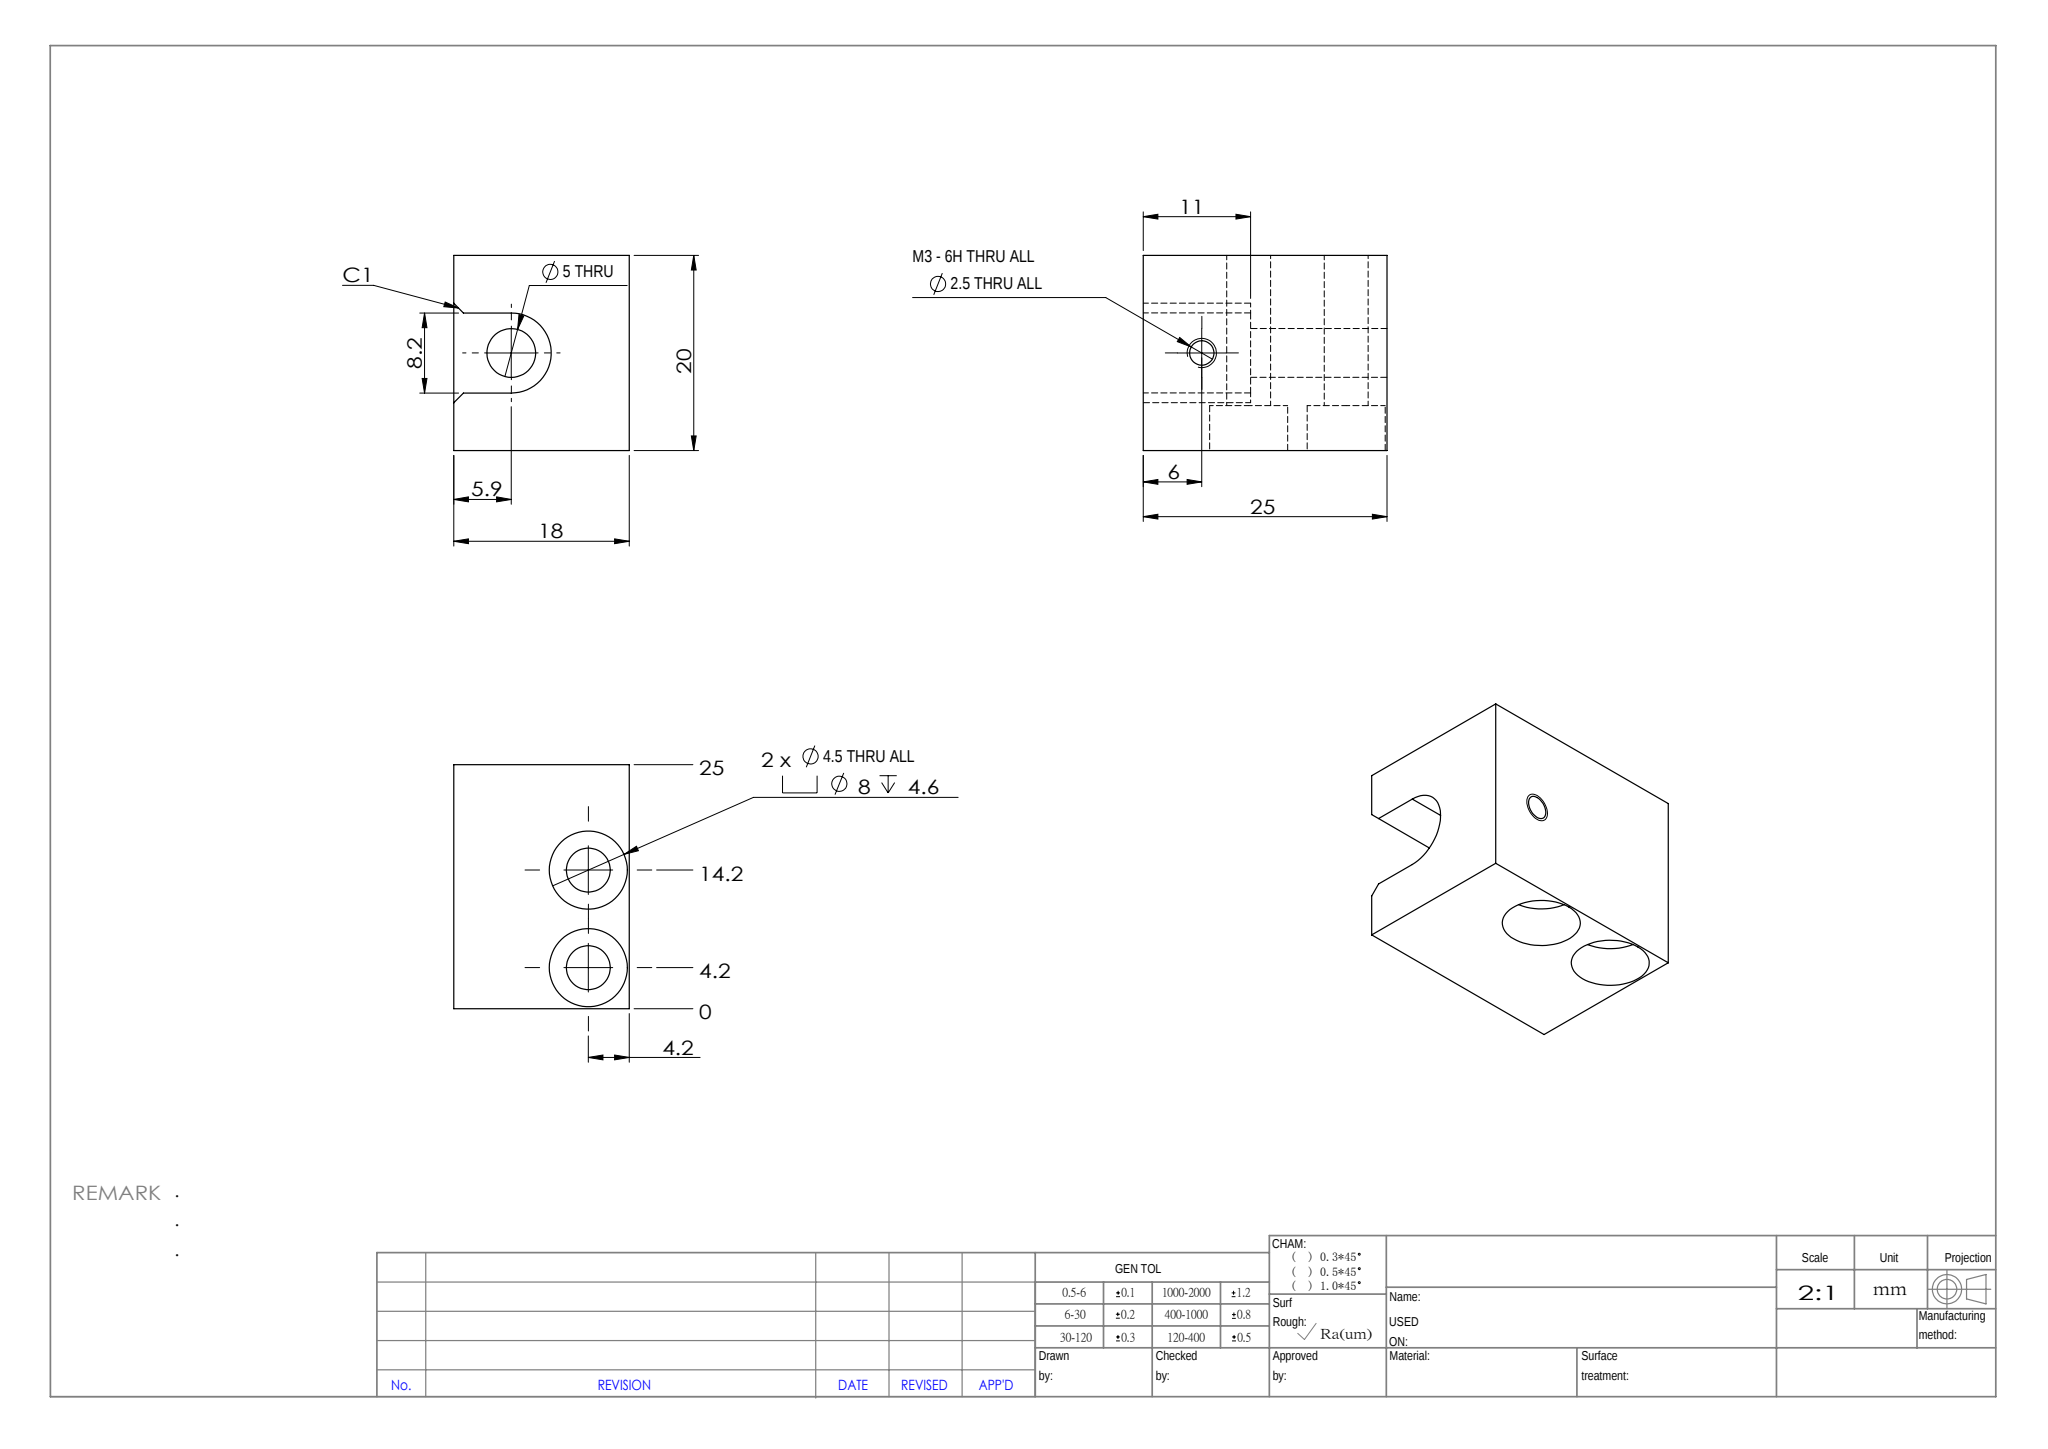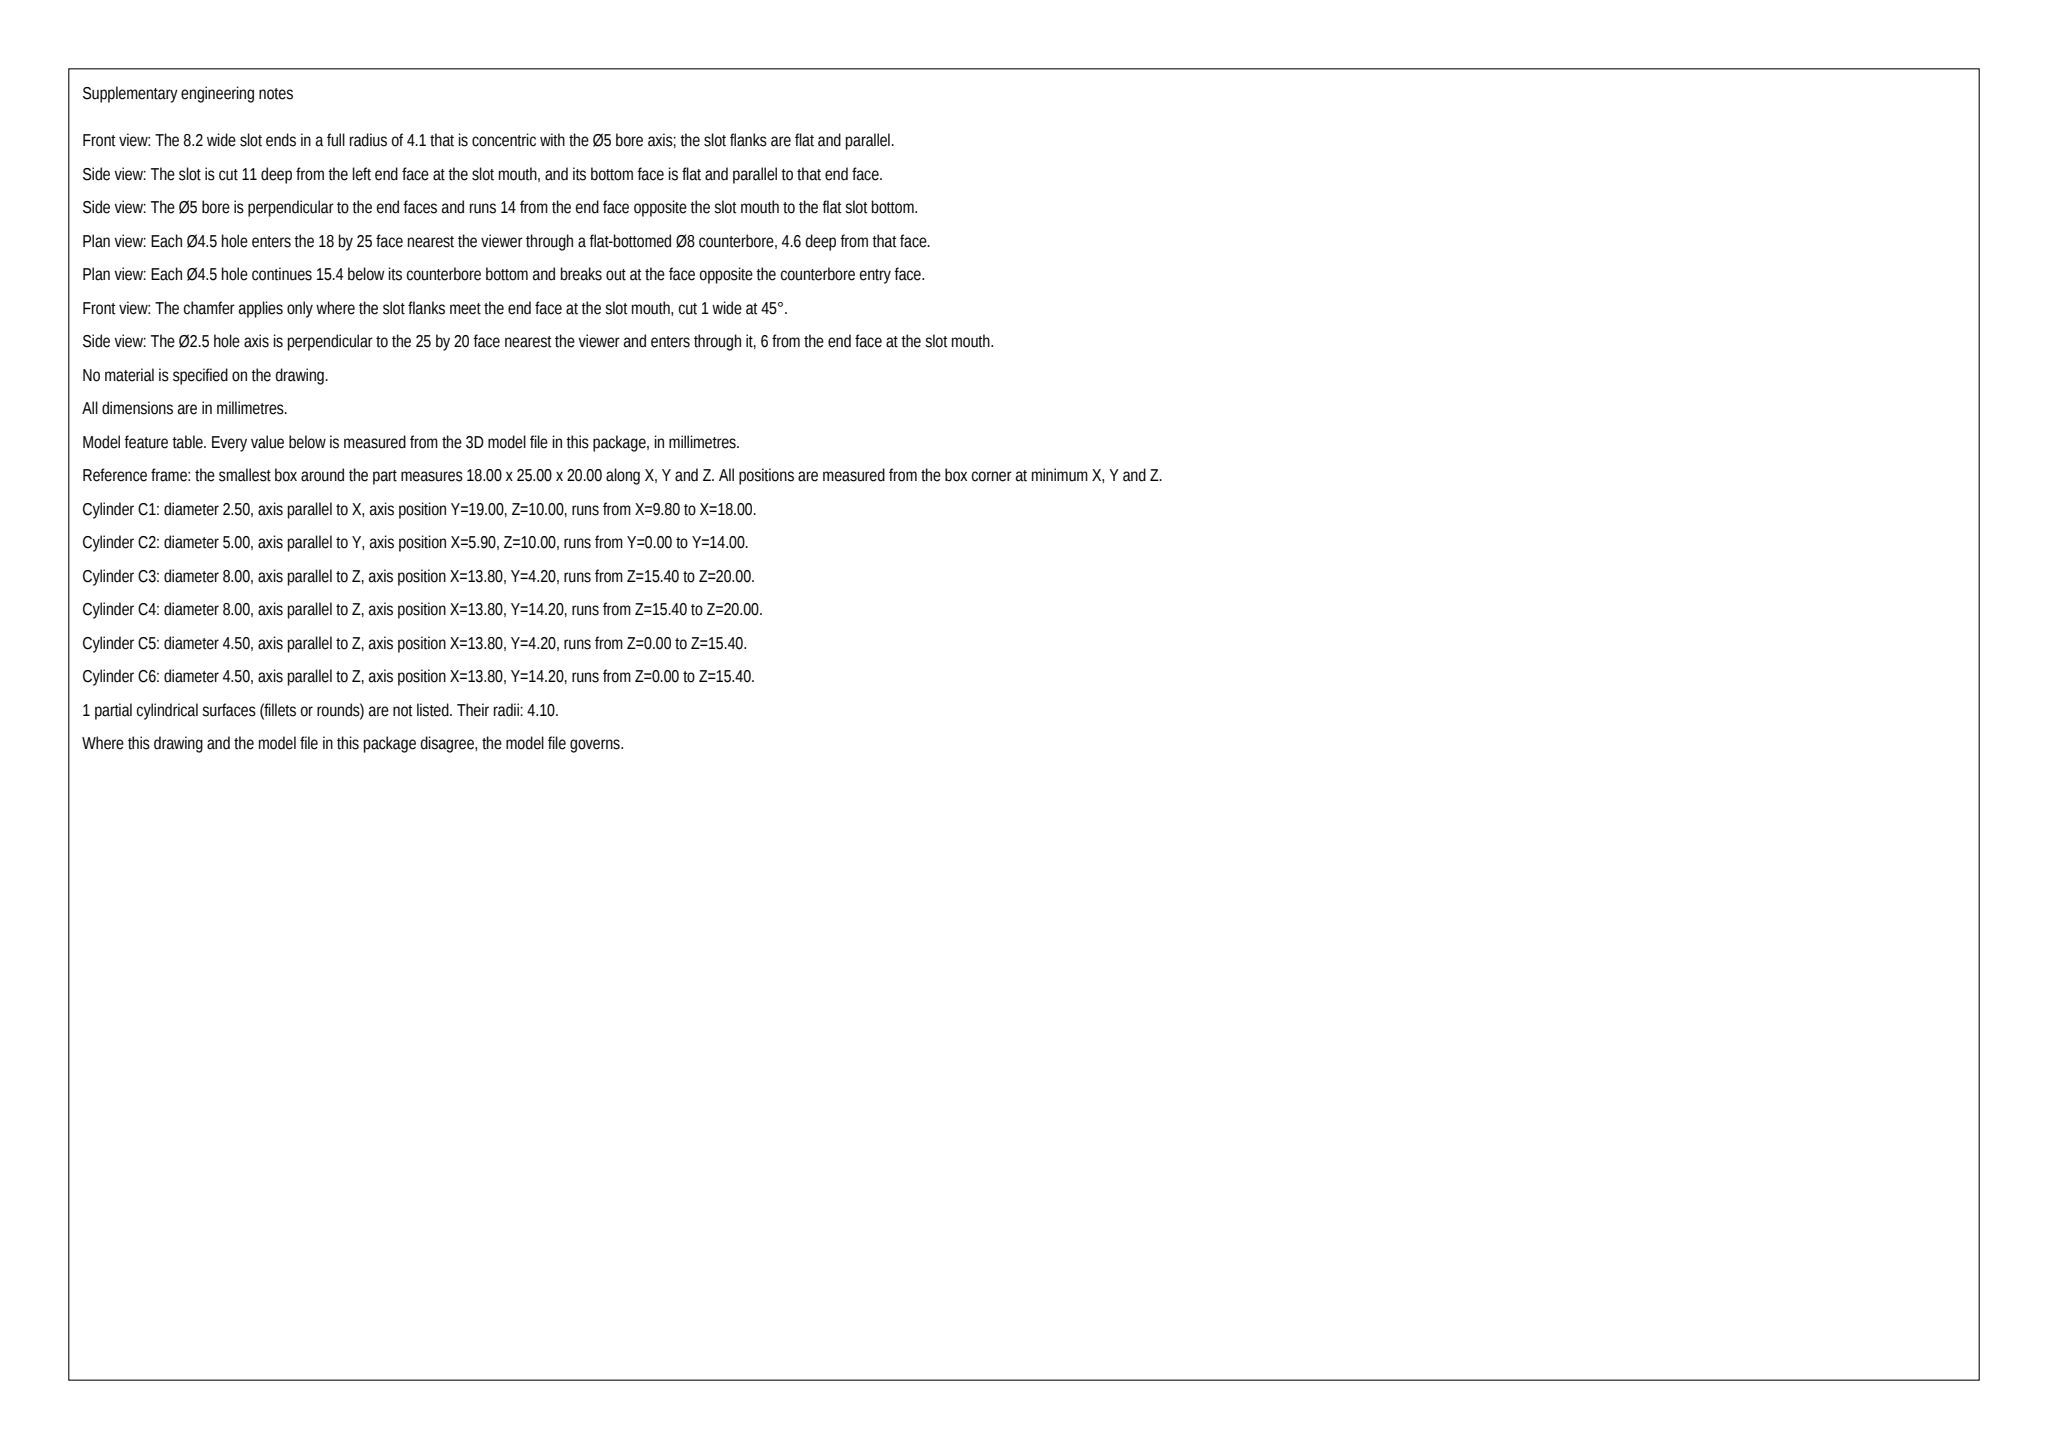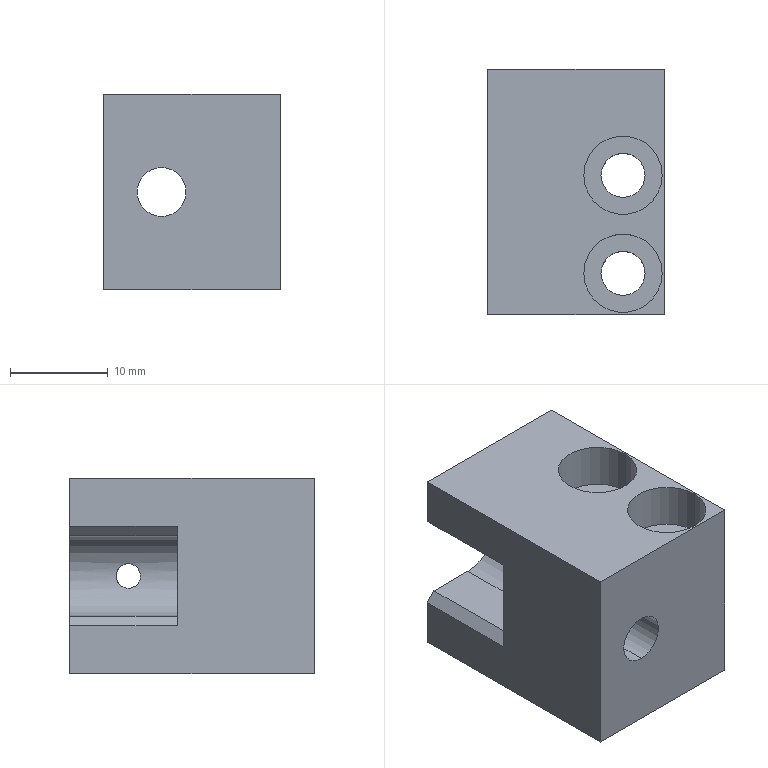Part | SolidWorks | mm | 1 solid | 26 faces | box 18 x 25 x 20 mm | volume 6900 mm3 | cylinder 13 | plane 13 | commonest cylinder face diameters 8 x4 4.5 x4 2.5 x2 5 x2 8.2 x1
Drawing notes:
FRONT VIEW: Ø5 THRU & Ø8.2 SLOT CL 10 ABOVE BASE | from the solid: Ø5 and Ø8.2 cyls, axis Y, pos z=10.0 of 20.0 bbox height
SIDE VIEW: M3-6H / Ø2.5 THRU CL 10 ABOVE BASE | from the solid: Ø2.5 cyl, axis X, pos z=10.0 from z=0 base face
2X Ø4.5 THRU, CBORE Ø8 DP 4.6 FROM TOP FACE (TOP VIEW) | from the solid: Ø8 cbore z-axis from z=15.4 to z=20.0; Ø4.5 z=0 to 15.4
STEP:
#1=CARTESIAN_POINT('',(0.8,14.2,5.4));
#2=VERTEX_POINT('',#1);
#3=CARTESIAN_POINT('',(8.8,14.2,5.4));
#4=VERTEX_POINT('',#3);
#5=CARTESIAN_POINT('',(4.8,14.2,5.4));
#6=DIRECTION('',(0.,0.,1.));
#7=DIRECTION('',(1.,0.,0.));
#8=AXIS2_PLACEMENT_3D('',#5,#6,#7);
#9=CIRCLE('',#8,4.);
#10=EDGE_CURVE('',#2,#4,#9,.T.);
#11=ORIENTED_EDGE('',*,*,#10,.F.);
#12=CARTESIAN_POINT('',(0.8,14.2,10.));
#13=VERTEX_POINT('',#12);
#14=CARTESIAN_POINT('',(0.8,14.2,10.));
#15=DIRECTION('',(0.,0.,1.));
#16=VECTOR('',#15,1000.);
#17=LINE('',#14,#16);
#18=EDGE_CURVE('',#2,#13,#17,.T.);
#19=ORIENTED_EDGE('',*,*,#18,.T.);
#20=CARTESIAN_POINT('',(8.8,14.2,10.));
#21=VERTEX_POINT('',#20);
#22=CARTESIAN_POINT('',(4.8,14.2,10.));
#23=DIRECTION('',(0.,0.,1.));
#24=DIRECTION('',(1.,0.,0.));
#25=AXIS2_PLACEMENT_3D('',#22,#23,#24);
#26=CIRCLE('',#25,4.);
#27=EDGE_CURVE('',#13,#21,#26,.T.);
#28=ORIENTED_EDGE('',*,*,#27,.T.);
#29=CARTESIAN_POINT('',(8.8,14.2,10.));
#30=DIRECTION('',(0.,0.,1.));
#31=VECTOR('',#30,1000.);
#32=LINE('',#29,#31);
#33=EDGE_CURVE('',#4,#21,#32,.T.);
#34=ORIENTED_EDGE('',*,*,#33,.F.);
#35=EDGE_LOOP('',(#11,#19,#28,#34));
#36=FACE_OUTER_BOUND('',#35,.T.);
#37=CARTESIAN_POINT('',(4.8,14.2,10.));
#38=DIRECTION('',(0.,0.,1.));
#39=DIRECTION('',(1.,0.,0.));
#40=AXIS2_PLACEMENT_3D('',#37,#38,#39);
#41=CYLINDRICAL_SURFACE('',#40,4.);
#42=ADVANCED_FACE('',(#36),#41,.F.);
#43=CARTESIAN_POINT('',(2.55,14.2,-10.));
#44=VERTEX_POINT('',#43);
#45=CARTESIAN_POINT('',(7.05,14.2,-10.));
#46=VERTEX_POINT('',#45);
#47=CARTESIAN_POINT('',(4.8,14.2,-10.));
#48=DIRECTION('',(0.,0.,1.));
#49=DIRECTION('',(1.,0.,0.));
#50=AXIS2_PLACEMENT_3D('',#47,#48,#49);
#51=CIRCLE('',#50,2.25);
#52=EDGE_CURVE('',#44,#46,#51,.T.);
#53=ORIENTED_EDGE('',*,*,#52,.F.);
#54=CARTESIAN_POINT('',(2.55,14.2,5.4));
#55=VERTEX_POINT('',#54);
#56=CARTESIAN_POINT('',(2.55,14.2,10.));
#57=DIRECTION('',(0.,0.,1.));
#58=VECTOR('',#57,1000.);
#59=LINE('',#56,#58);
#60=EDGE_CURVE('',#44,#55,#59,.T.);
#61=ORIENTED_EDGE('',*,*,#60,.T.);
#62=CARTESIAN_POINT('',(7.05,14.2,5.4));
#63=VERTEX_POINT('',#62);
#64=CARTESIAN_POINT('',(4.8,14.2,5.4));
#65=DIRECTION('',(0.,0.,1.));
#66=DIRECTION('',(1.,0.,0.));
#67=AXIS2_PLACEMENT_3D('',#64,#65,#66);
#68=CIRCLE('',#67,2.25);
#69=EDGE_CURVE('',#55,#63,#68,.T.);
#70=ORIENTED_EDGE('',*,*,#69,.T.);
#71=CARTESIAN_POINT('',(7.05,14.2,10.));
#72=DIRECTION('',(0.,0.,1.));
#73=VECTOR('',#72,1000.);
#74=LINE('',#71,#73);
#75=EDGE_CURVE('',#46,#63,#74,.T.);
#76=ORIENTED_EDGE('',*,*,#75,.F.);
#77=EDGE_LOOP('',(#53,#61,#70,#76));
#78=FACE_OUTER_BOUND('',#77,.T.);
#79=CARTESIAN_POINT('',(4.8,14.2,10.));
#80=DIRECTION('',(0.,0.,1.));
#81=DIRECTION('',(1.,0.,0.));
#82=AXIS2_PLACEMENT_3D('',#79,#80,#81);
#83=CYLINDRICAL_SURFACE('',#82,2.25);
#84=ADVANCED_FACE('',(#78),#83,.F.);
#85=CARTESIAN_POINT('',(0.8,4.2,5.4));
#86=VERTEX_POINT('',#85);
#87=CARTESIAN_POINT('',(8.8,4.2,5.4));
#88=VERTEX_POINT('',#87);
#89=CARTESIAN_POINT('',(4.8,4.2,5.4));
#90=DIRECTION('',(0.,0.,1.));
#91=DIRECTION('',(1.,0.,0.));
#92=AXIS2_PLACEMENT_3D('',#89,#90,#91);
#93=CIRCLE('',#92,4.);
#94=EDGE_CURVE('',#86,#88,#93,.T.);
#95=ORIENTED_EDGE('',*,*,#94,.F.);
#96=CARTESIAN_POINT('',(0.8,4.2,10.));
#97=VERTEX_POINT('',#96);
#98=CARTESIAN_POINT('',(0.8,4.2,10.));
#99=DIRECTION('',(0.,0.,1.));
#100=VECTOR('',#99,1000.);
#101=LINE('',#98,#100);
#102=EDGE_CURVE('',#86,#97,#101,.T.);
#103=ORIENTED_EDGE('',*,*,#102,.T.);
#104=CARTESIAN_POINT('',(8.8,4.2,10.));
#105=VERTEX_POINT('',#104);
#106=CARTESIAN_POINT('',(4.8,4.2,10.));
#107=DIRECTION('',(0.,0.,1.));
#108=DIRECTION('',(1.,0.,0.));
#109=AXIS2_PLACEMENT_3D('',#106,#107,#108);
#110=CIRCLE('',#109,4.);
#111=EDGE_CURVE('',#97,#105,#110,.T.);
#112=ORIENTED_EDGE('',*,*,#111,.T.);
#113=CARTESIAN_POINT('',(8.8,4.2,10.));
#114=DIRECTION('',(0.,0.,1.));
#115=VECTOR('',#114,1000.);
#116=LINE('',#113,#115);
#117=EDGE_CURVE('',#88,#105,#116,.T.);
#118=ORIENTED_EDGE('',*,*,#117,.F.);
#119=EDGE_LOOP('',(#95,#103,#112,#118));
#120=FACE_OUTER_BOUND('',#119,.T.);
#121=CARTESIAN_POINT('',(4.8,4.2,10.));
#122=DIRECTION('',(0.,0.,1.));
#123=DIRECTION('',(1.,0.,0.));
#124=AXIS2_PLACEMENT_3D('',#121,#122,#123);
#125=CYLINDRICAL_SURFACE('',#124,4.);
#126=ADVANCED_FACE('',(#120),#125,.F.);
#127=CARTESIAN_POINT('',(2.55,4.2,-10.));
#128=VERTEX_POINT('',#127);
#129=CARTESIAN_POINT('',(7.05,4.2,-10.));
#130=VERTEX_POINT('',#129);
#131=CARTESIAN_POINT('',(4.8,4.2,-10.));
#132=DIRECTION('',(0.,0.,1.));
#133=DIRECTION('',(1.,0.,0.));
#134=AXIS2_PLACEMENT_3D('',#131,#132,#133);
#135=CIRCLE('',#134,2.25);
#136=EDGE_CURVE('',#128,#130,#135,.T.);
#137=ORIENTED_EDGE('',*,*,#136,.F.);
#138=CARTESIAN_POINT('',(2.55,4.2,5.4));
#139=VERTEX_POINT('',#138);
#140=CARTESIAN_POINT('',(2.55,4.2,10.));
#141=DIRECTION('',(0.,0.,1.));
#142=VECTOR('',#141,1000.);
#143=LINE('',#140,#142);
#144=EDGE_CURVE('',#128,#139,#143,.T.);
#145=ORIENTED_EDGE('',*,*,#144,.T.);
#146=CARTESIAN_POINT('',(7.05,4.2,5.4));
#147=VERTEX_POINT('',#146);
#148=CARTESIAN_POINT('',(4.8,4.2,5.4));
#149=DIRECTION('',(0.,0.,1.));
#150=DIRECTION('',(1.,0.,0.));
#151=AXIS2_PLACEMENT_3D('',#148,#149,#150);
#152=CIRCLE('',#151,2.25);
#153=EDGE_CURVE('',#139,#147,#152,.T.);
#154=ORIENTED_EDGE('',*,*,#153,.T.);
#155=CARTESIAN_POINT('',(7.05,4.2,10.));
#156=DIRECTION('',(0.,0.,1.));
#157=VECTOR('',#156,1000.);
#158=LINE('',#155,#157);
#159=EDGE_CURVE('',#130,#147,#158,.T.);
#160=ORIENTED_EDGE('',*,*,#159,.F.);
#161=EDGE_LOOP('',(#137,#145,#154,#160));
#162=FACE_OUTER_BOUND('',#161,.T.);
#163=CARTESIAN_POINT('',(4.8,4.2,10.));
#164=DIRECTION('',(0.,0.,1.));
#165=DIRECTION('',(1.,0.,0.));
#166=AXIS2_PLACEMENT_3D('',#163,#164,#165);
#167=CYLINDRICAL_SURFACE('',#166,2.25);
#168=ADVANCED_FACE('',(#162),#167,.F.);
#169=CARTESIAN_POINT('',(0.8048,19.,1.25));
#170=VERTEX_POINT('',#169);
#171=CARTESIAN_POINT('',(0.8048,19.,-1.25));
#172=VERTEX_POINT('',#171);
#173=CARTESIAN_POINT('',(0.8048,19.,1.25));
#174=CARTESIAN_POINT('',(0.8048,18.836,1.25));
#175=CARTESIAN_POINT('',(0.8158,18.671,1.217));
#176=CARTESIAN_POINT('',(0.8525,18.37,1.092));
#177=CARTESIAN_POINT('',(0.8781,18.232,0.9994));
#178=CARTESIAN_POINT('',(0.929,18.001,0.7688));
#179=CARTESIAN_POINT('',(0.9538,17.909,0.6325));
#180=CARTESIAN_POINT('',(0.9898,17.783,0.3278));
#181=CARTESIAN_POINT('',(1.,17.75,0.1648));
#182=CARTESIAN_POINT('',(1.,17.75,-0.1647));
#183=CARTESIAN_POINT('',(0.9896,17.783,-0.3294));
#184=CARTESIAN_POINT('',(0.9541,17.908,-0.6306));
#185=CARTESIAN_POINT('',(0.9289,18.001,-0.7691));
#186=CARTESIAN_POINT('',(0.8783,18.231,-0.9983));
#187=CARTESIAN_POINT('',(0.8527,18.369,-1.091));
#188=CARTESIAN_POINT('',(0.8251,18.595,-1.185));
#189=CARTESIAN_POINT('',(0.8175,18.674,-1.21));
#190=CARTESIAN_POINT('',(0.8075,18.835,-1.242));
#191=CARTESIAN_POINT('',(0.8048,18.917,-1.25));
#192=CARTESIAN_POINT('',(0.8048,19.,-1.25));
#193=B_SPLINE_CURVE_WITH_KNOTS('',3,(#173,#174,#175,#176,#177,#178,#179,#180,#181,#182,#183,#184,#185,#186,#187,#188,#189,#190,#191,#192),.UNSPECIFIED.,.F.,.F.,(4,2,2,2,2,2,2,2,2,4),(0.003932,0.004423,0.004914,0.005405,0.005897,0.006388,0.006879,0.007371,0.007616,0.007862),.UNSPECIFIED.);
#194=EDGE_CURVE('',#170,#172,#193,.T.);
#195=ORIENTED_EDGE('',*,*,#194,.F.);
#196=CARTESIAN_POINT('',(9.,19.,1.25));
#197=VERTEX_POINT('',#196);
#198=CARTESIAN_POINT('',(9.,19.,1.25));
#199=DIRECTION('',(1.,0.,0.));
#200=VECTOR('',#199,1000.);
#201=LINE('',#198,#200);
#202=EDGE_CURVE('',#170,#197,#201,.T.);
#203=ORIENTED_EDGE('',*,*,#202,.T.);
#204=CARTESIAN_POINT('',(9.,19.,-1.25));
#205=VERTEX_POINT('',#204);
#206=CARTESIAN_POINT('',(9.,19.,0.));
#207=DIRECTION('',(1.,0.,0.));
#208=DIRECTION('',(0.,0.,-1.));
#209=AXIS2_PLACEMENT_3D('',#206,#207,#208);
#210=CIRCLE('',#209,1.25);
#211=EDGE_CURVE('',#197,#205,#210,.T.);
#212=ORIENTED_EDGE('',*,*,#211,.T.);
#213=CARTESIAN_POINT('',(9.,19.,-1.25));
#214=DIRECTION('',(1.,0.,0.));
#215=VECTOR('',#214,1000.);
#216=LINE('',#213,#215);
#217=EDGE_CURVE('',#172,#205,#216,.T.);
#218=ORIENTED_EDGE('',*,*,#217,.F.);
#219=EDGE_LOOP('',(#195,#203,#212,#218));
#220=FACE_OUTER_BOUND('',#219,.T.);
#221=CARTESIAN_POINT('',(9.,19.,0.));
#222=DIRECTION('',(1.,0.,0.));
#223=DIRECTION('',(0.,0.,-1.));
#224=AXIS2_PLACEMENT_3D('',#221,#222,#223);
#225=CYLINDRICAL_SURFACE('',#224,1.25);
#226=ADVANCED_FACE('',(#220),#225,.F.);
#227=CARTESIAN_POINT('',(-3.1,0.,-2.5));
#228=VERTEX_POINT('',#227);
#229=CARTESIAN_POINT('',(-3.1,0.,2.5));
#230=VERTEX_POINT('',#229);
#231=CARTESIAN_POINT('',(-3.1,0.,0.));
#232=DIRECTION('',(0.,1.,0.));
#233=DIRECTION('',(0.,0.,1.));
#234=AXIS2_PLACEMENT_3D('',#231,#232,#233);
#235=CIRCLE('',#234,2.5);
#236=EDGE_CURVE('',#228,#230,#235,.T.);
#237=ORIENTED_EDGE('',*,*,#236,.F.);
#238=CARTESIAN_POINT('',(-3.1,14.,-2.5));
#239=VERTEX_POINT('',#238);
#240=CARTESIAN_POINT('',(-3.1,0.,-2.5));
#241=DIRECTION('',(0.,1.,0.));
#242=VECTOR('',#241,1000.);
#243=LINE('',#240,#242);
#244=EDGE_CURVE('',#228,#239,#243,.T.);
#245=ORIENTED_EDGE('',*,*,#244,.T.);
#246=CARTESIAN_POINT('',(-3.1,14.,2.5));
#247=VERTEX_POINT('',#246);
#248=CARTESIAN_POINT('',(-3.1,14.,0.));
#249=DIRECTION('',(0.,1.,0.));
#250=DIRECTION('',(0.,0.,1.));
#251=AXIS2_PLACEMENT_3D('',#248,#249,#250);
#252=CIRCLE('',#251,2.5);
#253=EDGE_CURVE('',#239,#247,#252,.T.);
#254=ORIENTED_EDGE('',*,*,#253,.T.);
#255=CARTESIAN_POINT('',(-3.1,0.,2.5));
#256=DIRECTION('',(0.,1.,0.));
#257=VECTOR('',#256,1000.);
#258=LINE('',#255,#257);
#259=EDGE_CURVE('',#230,#247,#258,.T.);
#260=ORIENTED_EDGE('',*,*,#259,.F.);
#261=EDGE_LOOP('',(#237,#245,#254,#260));
#262=FACE_OUTER_BOUND('',#261,.T.);
#263=CARTESIAN_POINT('',(-3.1,0.,0.));
#264=DIRECTION('',(0.,1.,0.));
#265=DIRECTION('',(0.,0.,1.));
#266=AXIS2_PLACEMENT_3D('',#263,#264,#265);
#267=CYLINDRICAL_SURFACE('',#266,2.5);
#268=ADVANCED_FACE('',(#262),#267,.F.);
#269=CARTESIAN_POINT('',(-3.1,14.,0.));
#270=DIRECTION('',(0.,1.,0.));
#271=DIRECTION('',(0.,0.,1.));
#272=AXIS2_PLACEMENT_3D('',#269,#270,#271);
#273=CIRCLE('',#272,2.5);
#274=EDGE_CURVE('',#247,#239,#273,.T.);
#275=ORIENTED_EDGE('',*,*,#274,.F.);
#276=ORIENTED_EDGE('',*,*,#253,.F.);
#277=EDGE_LOOP('',(#275,#276));
#278=FACE_BOUND('',#277,.T.);
#279=CARTESIAN_POINT('',(-9.,14.,-5.1));
#280=VERTEX_POINT('',#279);
#281=CARTESIAN_POINT('',(-9.,14.,5.1));
#282=VERTEX_POINT('',#281);
#283=CARTESIAN_POINT('',(-9.,14.,-4.1));
#284=DIRECTION('',(0.,0.,1.));
#285=VECTOR('',#284,1000.);
#286=LINE('',#283,#285);
#287=EDGE_CURVE('',#280,#282,#286,.T.);
#288=ORIENTED_EDGE('',*,*,#287,.T.);
#289=CARTESIAN_POINT('',(-8.,14.,4.1));
#290=VERTEX_POINT('',#289);
#291=CARTESIAN_POINT('',(-8.,14.,4.1));
#292=DIRECTION('',(0.7071,0.,-0.7071));
#293=VECTOR('',#292,1000.);
#294=LINE('',#291,#293);
#295=EDGE_CURVE('',#282,#290,#294,.T.);
#296=ORIENTED_EDGE('',*,*,#295,.T.);
#297=CARTESIAN_POINT('',(-3.1,14.,4.1));
#298=VERTEX_POINT('',#297);
#299=CARTESIAN_POINT('',(-9.,14.,4.1));
#300=DIRECTION('',(1.,0.,0.));
#301=VECTOR('',#300,1000.);
#302=LINE('',#299,#301);
#303=EDGE_CURVE('',#290,#298,#302,.T.);
#304=ORIENTED_EDGE('',*,*,#303,.T.);
#305=CARTESIAN_POINT('',(-3.1,14.,-4.1));
#306=VERTEX_POINT('',#305);
#307=CARTESIAN_POINT('',(-3.1,14.,0.));
#308=DIRECTION('',(0.,-1.,0.));
#309=DIRECTION('',(0.,0.,1.));
#310=AXIS2_PLACEMENT_3D('',#307,#308,#309);
#311=CIRCLE('',#310,4.1);
#312=EDGE_CURVE('',#306,#298,#311,.T.);
#313=ORIENTED_EDGE('',*,*,#312,.F.);
#314=CARTESIAN_POINT('',(-8.,14.,-4.1));
#315=VERTEX_POINT('',#314);
#316=CARTESIAN_POINT('',(-9.,14.,-4.1));
#317=DIRECTION('',(-1.,0.,0.));
#318=VECTOR('',#317,1000.);
#319=LINE('',#316,#318);
#320=EDGE_CURVE('',#306,#315,#319,.T.);
#321=ORIENTED_EDGE('',*,*,#320,.T.);
#322=CARTESIAN_POINT('',(-9.,14.,-5.1));
#323=DIRECTION('',(-0.7071,0.,-0.7071));
#324=VECTOR('',#323,1000.);
#325=LINE('',#322,#324);
#326=EDGE_CURVE('',#315,#280,#325,.T.);
#327=ORIENTED_EDGE('',*,*,#326,.T.);
#328=EDGE_LOOP('',(#288,#296,#304,#313,#321,#327));
#329=FACE_OUTER_BOUND('',#328,.T.);
#330=CARTESIAN_POINT('',(0.,14.,0.));
#331=DIRECTION('',(0.,1.,0.));
#332=DIRECTION('',(0.,0.,1.));
#333=AXIS2_PLACEMENT_3D('',#330,#331,#332);
#334=PLANE('',#333);
#335=ADVANCED_FACE('',(#278,#329),#334,.T.);
#336=ORIENTED_EDGE('',*,*,#303,.F.);
#337=CARTESIAN_POINT('',(-8.,25.,4.1));
#338=VERTEX_POINT('',#337);
#339=CARTESIAN_POINT('',(-8.,14.,4.1));
#340=DIRECTION('',(0.,1.,0.));
#341=VECTOR('',#340,1000.);
#342=LINE('',#339,#341);
#343=EDGE_CURVE('',#290,#338,#342,.T.);
#344=ORIENTED_EDGE('',*,*,#343,.T.);
#345=CARTESIAN_POINT('',(-3.1,25.,4.1));
#346=VERTEX_POINT('',#345);
#347=CARTESIAN_POINT('',(-9.,25.,4.1));
#348=DIRECTION('',(1.,0.,0.));
#349=VECTOR('',#348,1000.);
#350=LINE('',#347,#349);
#351=EDGE_CURVE('',#338,#346,#350,.T.);
#352=ORIENTED_EDGE('',*,*,#351,.T.);
#353=CARTESIAN_POINT('',(-3.1,8.202,4.1));
#354=DIRECTION('',(0.,1.,0.));
#355=VECTOR('',#354,1000.);
#356=LINE('',#353,#355);
#357=EDGE_CURVE('',#298,#346,#356,.T.);
#358=ORIENTED_EDGE('',*,*,#357,.F.);
#359=EDGE_LOOP('',(#336,#344,#352,#358));
#360=FACE_OUTER_BOUND('',#359,.T.);
#361=CARTESIAN_POINT('',(-9.,14.,4.1));
#362=DIRECTION('',(0.,0.,1.));
#363=DIRECTION('',(1.,0.,0.));
#364=AXIS2_PLACEMENT_3D('',#361,#362,#363);
#365=PLANE('',#364);
#366=ADVANCED_FACE('',(#360),#365,.F.);
#367=CARTESIAN_POINT('',(9.,19.,0.));
#368=DIRECTION('',(1.,0.,0.));
#369=DIRECTION('',(0.,0.,-1.));
#370=AXIS2_PLACEMENT_3D('',#367,#368,#369);
#371=CIRCLE('',#370,1.25);
#372=EDGE_CURVE('',#205,#197,#371,.T.);
#373=ORIENTED_EDGE('',*,*,#372,.F.);
#374=ORIENTED_EDGE('',*,*,#211,.F.);
#375=EDGE_LOOP('',(#373,#374));
#376=FACE_BOUND('',#375,.T.);
#377=CARTESIAN_POINT('',(9.,0.,10.));
#378=VERTEX_POINT('',#377);
#379=CARTESIAN_POINT('',(9.,0.,-10.));
#380=VERTEX_POINT('',#379);
#381=CARTESIAN_POINT('',(9.,0.,10.));
#382=DIRECTION('',(0.,0.,-1.));
#383=VECTOR('',#382,1000.);
#384=LINE('',#381,#383);
#385=EDGE_CURVE('',#378,#380,#384,.T.);
#386=ORIENTED_EDGE('',*,*,#385,.T.);
#387=CARTESIAN_POINT('',(9.,25.,-10.));
#388=VERTEX_POINT('',#387);
#389=CARTESIAN_POINT('',(9.,25.,-10.));
#390=DIRECTION('',(0.,-1.,0.));
#391=VECTOR('',#390,1000.);
#392=LINE('',#389,#391);
#393=EDGE_CURVE('',#388,#380,#392,.T.);
#394=ORIENTED_EDGE('',*,*,#393,.F.);
#395=CARTESIAN_POINT('',(9.,25.,10.));
#396=VERTEX_POINT('',#395);
#397=CARTESIAN_POINT('',(9.,25.,10.));
#398=DIRECTION('',(0.,0.,-1.));
#399=VECTOR('',#398,1000.);
#400=LINE('',#397,#399);
#401=EDGE_CURVE('',#396,#388,#400,.T.);
#402=ORIENTED_EDGE('',*,*,#401,.F.);
#403=CARTESIAN_POINT('',(9.,25.,10.));
#404=DIRECTION('',(0.,-1.,0.));
#405=VECTOR('',#404,1000.);
#406=LINE('',#403,#405);
#407=EDGE_CURVE('',#396,#378,#406,.T.);
#408=ORIENTED_EDGE('',*,*,#407,.T.);
#409=EDGE_LOOP('',(#386,#394,#402,#408));
#410=FACE_OUTER_BOUND('',#409,.T.);
#411=CARTESIAN_POINT('',(9.,25.,10.));
#412=DIRECTION('',(-1.,0.,0.));
#413=DIRECTION('',(0.,0.,1.));
#414=AXIS2_PLACEMENT_3D('',#411,#412,#413);
#415=PLANE('',#414);
#416=ADVANCED_FACE('',(#376,#410),#415,.F.);
#417=CARTESIAN_POINT('',(4.8,14.2,-10.));
#418=DIRECTION('',(0.,0.,1.));
#419=DIRECTION('',(1.,0.,0.));
#420=AXIS2_PLACEMENT_3D('',#417,#418,#419);
#421=CIRCLE('',#420,2.25);
#422=EDGE_CURVE('',#46,#44,#421,.T.);
#423=ORIENTED_EDGE('',*,*,#422,.T.);
#424=ORIENTED_EDGE('',*,*,#52,.T.);
#425=EDGE_LOOP('',(#423,#424));
#426=FACE_BOUND('',#425,.T.);
#427=CARTESIAN_POINT('',(4.8,4.2,-10.));
#428=DIRECTION('',(0.,0.,1.));
#429=DIRECTION('',(1.,0.,0.));
#430=AXIS2_PLACEMENT_3D('',#427,#428,#429);
#431=CIRCLE('',#430,2.25);
#432=EDGE_CURVE('',#130,#128,#431,.T.);
#433=ORIENTED_EDGE('',*,*,#432,.T.);
#434=ORIENTED_EDGE('',*,*,#136,.T.);
#435=EDGE_LOOP('',(#433,#434));
#436=FACE_BOUND('',#435,.T.);
#437=CARTESIAN_POINT('',(-9.,0.,-10.));
#438=VERTEX_POINT('',#437);
#439=CARTESIAN_POINT('',(-9.,0.,-10.));
#440=DIRECTION('',(-1.,0.,0.));
#441=VECTOR('',#440,1000.);
#442=LINE('',#439,#441);
#443=EDGE_CURVE('',#380,#438,#442,.T.);
#444=ORIENTED_EDGE('',*,*,#443,.T.);
#445=CARTESIAN_POINT('',(-9.,25.,-10.));
#446=VERTEX_POINT('',#445);
#447=CARTESIAN_POINT('',(-9.,25.,-10.));
#448=DIRECTION('',(0.,-1.,0.));
#449=VECTOR('',#448,1000.);
#450=LINE('',#447,#449);
#451=EDGE_CURVE('',#446,#438,#450,.T.);
#452=ORIENTED_EDGE('',*,*,#451,.F.);
#453=CARTESIAN_POINT('',(-9.,25.,-10.));
#454=DIRECTION('',(-1.,0.,0.));
#455=VECTOR('',#454,1000.);
#456=LINE('',#453,#455);
#457=EDGE_CURVE('',#388,#446,#456,.T.);
#458=ORIENTED_EDGE('',*,*,#457,.F.);
#459=ORIENTED_EDGE('',*,*,#393,.T.);
#460=EDGE_LOOP('',(#444,#452,#458,#459));
#461=FACE_OUTER_BOUND('',#460,.T.);
#462=CARTESIAN_POINT('',(-9.,25.,-10.));
#463=DIRECTION('',(0.,0.,1.));
#464=DIRECTION('',(1.,0.,0.));
#465=AXIS2_PLACEMENT_3D('',#462,#463,#464);
#466=PLANE('',#465);
#467=ADVANCED_FACE('',(#426,#436,#461),#466,.F.);
#468=CARTESIAN_POINT('',(-9.,25.,5.1));
#469=VERTEX_POINT('',#468);
#470=CARTESIAN_POINT('',(-9.,25.,10.));
#471=VERTEX_POINT('',#470);
#472=CARTESIAN_POINT('',(-9.,25.,10.));
#473=DIRECTION('',(0.,0.,1.));
#474=VECTOR('',#473,1000.);
#475=LINE('',#472,#474);
#476=EDGE_CURVE('',#469,#471,#475,.T.);
#477=ORIENTED_EDGE('',*,*,#476,.F.);
#478=CARTESIAN_POINT('',(-9.,25.,5.1));
#479=DIRECTION('',(0.,-1.,0.));
#480=VECTOR('',#479,1000.);
#481=LINE('',#478,#480);
#482=EDGE_CURVE('',#469,#282,#481,.T.);
#483=ORIENTED_EDGE('',*,*,#482,.T.);
#484=ORIENTED_EDGE('',*,*,#287,.F.);
#485=CARTESIAN_POINT('',(-9.,25.,-5.1));
#486=VERTEX_POINT('',#485);
#487=CARTESIAN_POINT('',(-9.,25.,-5.1));
#488=DIRECTION('',(0.,1.,0.));
#489=VECTOR('',#488,1000.);
#490=LINE('',#487,#489);
#491=EDGE_CURVE('',#280,#486,#490,.T.);
#492=ORIENTED_EDGE('',*,*,#491,.T.);
#493=CARTESIAN_POINT('',(-9.,25.,10.));
#494=DIRECTION('',(0.,0.,1.));
#495=VECTOR('',#494,1000.);
#496=LINE('',#493,#495);
#497=EDGE_CURVE('',#446,#486,#496,.T.);
#498=ORIENTED_EDGE('',*,*,#497,.F.);
#499=ORIENTED_EDGE('',*,*,#451,.T.);
#500=CARTESIAN_POINT('',(-9.,0.,10.));
#501=VERTEX_POINT('',#500);
#502=CARTESIAN_POINT('',(-9.,0.,10.));
#503=DIRECTION('',(0.,0.,1.));
#504=VECTOR('',#503,1000.);
#505=LINE('',#502,#504);
#506=EDGE_CURVE('',#438,#501,#505,.T.);
#507=ORIENTED_EDGE('',*,*,#506,.T.);
#508=CARTESIAN_POINT('',(-9.,25.,10.));
#509=DIRECTION('',(0.,-1.,0.));
#510=VECTOR('',#509,1000.);
#511=LINE('',#508,#510);
#512=EDGE_CURVE('',#471,#501,#511,.T.);
#513=ORIENTED_EDGE('',*,*,#512,.F.);
#514=EDGE_LOOP('',(#477,#483,#484,#492,#498,#499,#507,#513));
#515=FACE_OUTER_BOUND('',#514,.T.);
#516=CARTESIAN_POINT('',(-9.,25.,10.));
#517=DIRECTION('',(1.,0.,0.));
#518=DIRECTION('',(0.,0.,-1.));
#519=AXIS2_PLACEMENT_3D('',#516,#517,#518);
#520=PLANE('',#519);
#521=ADVANCED_FACE('',(#515),#520,.F.);
#522=CARTESIAN_POINT('',(4.8,14.2,10.));
#523=DIRECTION('',(0.,0.,1.));
#524=DIRECTION('',(1.,0.,0.));
#525=AXIS2_PLACEMENT_3D('',#522,#523,#524);
#526=CIRCLE('',#525,4.);
#527=EDGE_CURVE('',#21,#13,#526,.T.);
#528=ORIENTED_EDGE('',*,*,#527,.F.);
#529=ORIENTED_EDGE('',*,*,#27,.F.);
#530=EDGE_LOOP('',(#528,#529));
#531=FACE_BOUND('',#530,.T.);
#532=CARTESIAN_POINT('',(4.8,4.2,10.));
#533=DIRECTION('',(0.,0.,1.));
#534=DIRECTION('',(1.,0.,0.));
#535=AXIS2_PLACEMENT_3D('',#532,#533,#534);
#536=CIRCLE('',#535,4.);
#537=EDGE_CURVE('',#105,#97,#536,.T.);
#538=ORIENTED_EDGE('',*,*,#537,.F.);
#539=ORIENTED_EDGE('',*,*,#111,.F.);
#540=EDGE_LOOP('',(#538,#539));
#541=FACE_BOUND('',#540,.T.);
#542=CARTESIAN_POINT('',(-9.,0.,10.));
#543=DIRECTION('',(1.,0.,0.));
#544=VECTOR('',#543,1000.);
#545=LINE('',#542,#544);
#546=EDGE_CURVE('',#501,#378,#545,.T.);
#547=ORIENTED_EDGE('',*,*,#546,.T.);
#548=ORIENTED_EDGE('',*,*,#407,.F.);
#549=CARTESIAN_POINT('',(-9.,25.,10.));
#550=DIRECTION('',(1.,0.,0.));
#551=VECTOR('',#550,1000.);
#552=LINE('',#549,#551);
#553=EDGE_CURVE('',#471,#396,#552,.T.);
#554=ORIENTED_EDGE('',*,*,#553,.F.);
#555=ORIENTED_EDGE('',*,*,#512,.T.);
#556=EDGE_LOOP('',(#547,#548,#554,#555));
#557=FACE_OUTER_BOUND('',#556,.T.);
#558=CARTESIAN_POINT('',(-9.,25.,10.));
#559=DIRECTION('',(0.,0.,-1.));
#560=DIRECTION('',(-1.,0.,0.));
#561=AXIS2_PLACEMENT_3D('',#558,#559,#560);
#562=PLANE('',#561);
#563=ADVANCED_FACE('',(#531,#541,#557),#562,.F.);
#564=ORIENTED_EDGE('',*,*,#351,.F.);
#565=CARTESIAN_POINT('',(-8.,25.,4.1));
#566=DIRECTION('',(-0.7071,0.,0.7071));
#567=VECTOR('',#566,1000.);
#568=LINE('',#565,#567);
#569=EDGE_CURVE('',#338,#469,#568,.T.);
#570=ORIENTED_EDGE('',*,*,#569,.T.);
#571=ORIENTED_EDGE('',*,*,#476,.T.);
#572=ORIENTED_EDGE('',*,*,#553,.T.);
#573=ORIENTED_EDGE('',*,*,#401,.T.);
#574=ORIENTED_EDGE('',*,*,#457,.T.);
#575=ORIENTED_EDGE('',*,*,#497,.T.);
#576=CARTESIAN_POINT('',(-8.,25.,-4.1));
#577=VERTEX_POINT('',#576);
#578=CARTESIAN_POINT('',(-9.,25.,-5.1));
#579=DIRECTION('',(0.7071,0.,0.7071));
#580=VECTOR('',#579,1000.);
#581=LINE('',#578,#580);
#582=EDGE_CURVE('',#486,#577,#581,.T.);
#583=ORIENTED_EDGE('',*,*,#582,.T.);
#584=CARTESIAN_POINT('',(-3.1,25.,-4.1));
#585=VERTEX_POINT('',#584);
#586=CARTESIAN_POINT('',(-9.,25.,-4.1));
#587=DIRECTION('',(-1.,0.,0.));
#588=VECTOR('',#587,1000.);
#589=LINE('',#586,#588);
#590=EDGE_CURVE('',#585,#577,#589,.T.);
#591=ORIENTED_EDGE('',*,*,#590,.F.);
#592=CARTESIAN_POINT('',(-3.1,25.,0.));
#593=DIRECTION('',(0.,1.,0.));
#594=DIRECTION('',(0.,0.,1.));
#595=AXIS2_PLACEMENT_3D('',#592,#593,#594);
#596=CIRCLE('',#595,4.1);
#597=EDGE_CURVE('',#346,#585,#596,.T.);
#598=ORIENTED_EDGE('',*,*,#597,.F.);
#599=EDGE_LOOP('',(#564,#570,#571,#572,#573,#574,#575,#583,#591,#598));
#600=FACE_OUTER_BOUND('',#599,.T.);
#601=CARTESIAN_POINT('',(0.,25.,0.));
#602=DIRECTION('',(0.,-1.,0.));
#603=DIRECTION('',(0.,0.,-1.));
#604=AXIS2_PLACEMENT_3D('',#601,#602,#603);
#605=PLANE('',#604);
#606=ADVANCED_FACE('',(#600),#605,.F.);
#607=CARTESIAN_POINT('',(-3.1,0.,0.));
#608=DIRECTION('',(0.,1.,0.));
#609=DIRECTION('',(0.,0.,1.));
#610=AXIS2_PLACEMENT_3D('',#607,#608,#609);
#611=CIRCLE('',#610,2.5);
#612=EDGE_CURVE('',#230,#228,#611,.T.);
#613=ORIENTED_EDGE('',*,*,#612,.T.);
#614=ORIENTED_EDGE('',*,*,#236,.T.);
#615=EDGE_LOOP('',(#613,#614));
#616=FACE_BOUND('',#615,.T.);
#617=ORIENTED_EDGE('',*,*,#385,.F.);
#618=ORIENTED_EDGE('',*,*,#546,.F.);
#619=ORIENTED_EDGE('',*,*,#506,.F.);
#620=ORIENTED_EDGE('',*,*,#443,.F.);
#621=EDGE_LOOP('',(#617,#618,#619,#620));
#622=FACE_OUTER_BOUND('',#621,.T.);
#623=CARTESIAN_POINT('',(0.,0.,0.));
#624=DIRECTION('',(0.,-1.,0.));
#625=DIRECTION('',(0.,0.,-1.));
#626=AXIS2_PLACEMENT_3D('',#623,#624,#625);
#627=PLANE('',#626);
#628=ADVANCED_FACE('',(#616,#622),#627,.T.);
#629=ORIENTED_EDGE('',*,*,#590,.T.);
#630=CARTESIAN_POINT('',(-8.,14.,-4.1));
#631=DIRECTION('',(0.,-1.,0.));
#632=VECTOR('',#631,1000.);
#633=LINE('',#630,#632);
#634=EDGE_CURVE('',#577,#315,#633,.T.);
#635=ORIENTED_EDGE('',*,*,#634,.T.);
#636=ORIENTED_EDGE('',*,*,#320,.F.);
#637=CARTESIAN_POINT('',(-3.1,8.202,-4.1));
#638=DIRECTION('',(0.,1.,0.));
#639=VECTOR('',#638,1000.);
#640=LINE('',#637,#639);
#641=EDGE_CURVE('',#306,#585,#640,.T.);
#642=ORIENTED_EDGE('',*,*,#641,.T.);
#643=EDGE_LOOP('',(#629,#635,#636,#642));
#644=FACE_OUTER_BOUND('',#643,.T.);
#645=CARTESIAN_POINT('',(-9.,14.,-4.1));
#646=DIRECTION('',(-0.,0.,-1.));
#647=DIRECTION('',(-1.,0.,0.));
#648=AXIS2_PLACEMENT_3D('',#645,#646,#647);
#649=PLANE('',#648);
#650=ADVANCED_FACE('',(#644),#649,.F.);
#651=CARTESIAN_POINT('',(0.8048,19.,-1.25));
#652=CARTESIAN_POINT('',(0.8048,19.166,-1.25));
#653=CARTESIAN_POINT('',(0.8158,19.329,-1.217));
#654=CARTESIAN_POINT('',(0.8527,19.632,-1.091));
#655=CARTESIAN_POINT('',(0.8783,19.77,-0.9983));
#656=CARTESIAN_POINT('',(0.9289,19.999,-0.7691));
#657=CARTESIAN_POINT('',(0.9541,20.092,-0.6304));
#658=CARTESIAN_POINT('',(0.9895,20.217,-0.3299));
#659=CARTESIAN_POINT('',(1.,20.25,-0.1647));
#660=CARTESIAN_POINT('',(1.,20.25,0.08155));
#661=CARTESIAN_POINT('',(0.9975,20.242,0.1649));
#662=CARTESIAN_POINT('',(0.9878,20.21,0.3257));
#663=CARTESIAN_POINT('',(0.9808,20.186,0.4039));
#664=CARTESIAN_POINT('',(0.9539,20.091,0.6319));
#665=CARTESIAN_POINT('',(0.929,19.999,0.7691));
#666=CARTESIAN_POINT('',(0.8908,19.826,0.942));
#667=CARTESIAN_POINT('',(0.8781,19.763,0.9934));
#668=CARTESIAN_POINT('',(0.8544,19.628,1.084));
#669=CARTESIAN_POINT('',(0.8433,19.555,1.123));
#670=CARTESIAN_POINT('',(0.8158,19.329,1.217));
#671=CARTESIAN_POINT('',(0.8048,19.164,1.25));
#672=CARTESIAN_POINT('',(0.8048,19.,1.25));
#673=B_SPLINE_CURVE_WITH_KNOTS('',3,(#651,#652,#653,#654,#655,#656,#657,#658,#659,#660,#661,#662,#663,#664,#665,#666,#667,#668,#669,#670,#671,#672),.UNSPECIFIED.,.F.,.F.,(4,2,2,2,2,2,2,2,2,2,4),(0.,0.0004914,0.0009829,0.001474,0.001966,0.002211,0.002457,0.002949,0.003194,0.00344,0.003932),.UNSPECIFIED.);
#674=EDGE_CURVE('',#172,#170,#673,.T.);
#675=ORIENTED_EDGE('',*,*,#674,.T.);
#676=ORIENTED_EDGE('',*,*,#194,.T.);
#677=EDGE_LOOP('',(#675,#676));
#678=FACE_BOUND('',#677,.T.);
#679=ORIENTED_EDGE('',*,*,#641,.F.);
#680=ORIENTED_EDGE('',*,*,#312,.T.);
#681=ORIENTED_EDGE('',*,*,#357,.T.);
#682=ORIENTED_EDGE('',*,*,#597,.T.);
#683=EDGE_LOOP('',(#679,#680,#681,#682));
#684=FACE_OUTER_BOUND('',#683,.T.);
#685=CARTESIAN_POINT('',(-3.1,8.202,0.));
#686=DIRECTION('',(0.,1.,0.));
#687=DIRECTION('',(0.,0.,1.));
#688=AXIS2_PLACEMENT_3D('',#685,#686,#687);
#689=CYLINDRICAL_SURFACE('',#688,4.1);
#690=ADVANCED_FACE('',(#678,#684),#689,.F.);
#691=ORIENTED_EDGE('',*,*,#244,.F.);
#692=ORIENTED_EDGE('',*,*,#612,.F.);
#693=ORIENTED_EDGE('',*,*,#259,.T.);
#694=ORIENTED_EDGE('',*,*,#274,.T.);
#695=EDGE_LOOP('',(#691,#692,#693,#694));
#696=FACE_OUTER_BOUND('',#695,.T.);
#697=CARTESIAN_POINT('',(-3.1,0.,0.));
#698=DIRECTION('',(0.,1.,0.));
#699=DIRECTION('',(0.,0.,1.));
#700=AXIS2_PLACEMENT_3D('',#697,#698,#699);
#701=CYLINDRICAL_SURFACE('',#700,2.5);
#702=ADVANCED_FACE('',(#696),#701,.F.);
#703=ORIENTED_EDGE('',*,*,#295,.F.);
#704=ORIENTED_EDGE('',*,*,#482,.F.);
#705=ORIENTED_EDGE('',*,*,#569,.F.);
#706=ORIENTED_EDGE('',*,*,#343,.F.);
#707=EDGE_LOOP('',(#703,#704,#705,#706));
#708=FACE_OUTER_BOUND('',#707,.T.);
#709=CARTESIAN_POINT('',(-8.,14.,4.1));
#710=DIRECTION('',(0.7071,0.,0.7071));
#711=DIRECTION('',(0.,1.,0.));
#712=AXIS2_PLACEMENT_3D('',#709,#710,#711);
#713=PLANE('',#712);
#714=ADVANCED_FACE('',(#708),#713,.F.);
#715=ORIENTED_EDGE('',*,*,#326,.F.);
#716=ORIENTED_EDGE('',*,*,#634,.F.);
#717=ORIENTED_EDGE('',*,*,#582,.F.);
#718=ORIENTED_EDGE('',*,*,#491,.F.);
#719=EDGE_LOOP('',(#715,#716,#717,#718));
#720=FACE_OUTER_BOUND('',#719,.T.);
#721=CARTESIAN_POINT('',(-9.,25.,-5.1));
#722=DIRECTION('',(0.7071,0.,-0.7071));
#723=DIRECTION('',(0.,1.,0.));
#724=AXIS2_PLACEMENT_3D('',#721,#722,#723);
#725=PLANE('',#724);
#726=ADVANCED_FACE('',(#720),#725,.F.);
#727=ORIENTED_EDGE('',*,*,#202,.F.);
#728=ORIENTED_EDGE('',*,*,#674,.F.);
#729=ORIENTED_EDGE('',*,*,#217,.T.);
#730=ORIENTED_EDGE('',*,*,#372,.T.);
#731=EDGE_LOOP('',(#727,#728,#729,#730));
#732=FACE_OUTER_BOUND('',#731,.T.);
#733=CARTESIAN_POINT('',(9.,19.,0.));
#734=DIRECTION('',(1.,0.,0.));
#735=DIRECTION('',(0.,0.,-1.));
#736=AXIS2_PLACEMENT_3D('',#733,#734,#735);
#737=CYLINDRICAL_SURFACE('',#736,1.25);
#738=ADVANCED_FACE('',(#732),#737,.F.);
#739=ORIENTED_EDGE('',*,*,#144,.F.);
#740=ORIENTED_EDGE('',*,*,#432,.F.);
#741=ORIENTED_EDGE('',*,*,#159,.T.);
#742=CARTESIAN_POINT('',(4.8,4.2,5.4));
#743=DIRECTION('',(0.,0.,1.));
#744=DIRECTION('',(1.,0.,0.));
#745=AXIS2_PLACEMENT_3D('',#742,#743,#744);
#746=CIRCLE('',#745,2.25);
#747=EDGE_CURVE('',#147,#139,#746,.T.);
#748=ORIENTED_EDGE('',*,*,#747,.T.);
#749=EDGE_LOOP('',(#739,#740,#741,#748));
#750=FACE_OUTER_BOUND('',#749,.T.);
#751=CARTESIAN_POINT('',(4.8,4.2,10.));
#752=DIRECTION('',(0.,0.,1.));
#753=DIRECTION('',(1.,0.,0.));
#754=AXIS2_PLACEMENT_3D('',#751,#752,#753);
#755=CYLINDRICAL_SURFACE('',#754,2.25);
#756=ADVANCED_FACE('',(#750),#755,.F.);
#757=ORIENTED_EDGE('',*,*,#747,.F.);
#758=ORIENTED_EDGE('',*,*,#153,.F.);
#759=EDGE_LOOP('',(#757,#758));
#760=FACE_BOUND('',#759,.T.);
#761=CARTESIAN_POINT('',(4.8,4.2,5.4));
#762=DIRECTION('',(0.,0.,1.));
#763=DIRECTION('',(1.,0.,0.));
#764=AXIS2_PLACEMENT_3D('',#761,#762,#763);
#765=CIRCLE('',#764,4.);
#766=EDGE_CURVE('',#88,#86,#765,.T.);
#767=ORIENTED_EDGE('',*,*,#766,.T.);
#768=ORIENTED_EDGE('',*,*,#94,.T.);
#769=EDGE_LOOP('',(#767,#768));
#770=FACE_OUTER_BOUND('',#769,.T.);
#771=CARTESIAN_POINT('',(7.05,4.2,5.4));
#772=DIRECTION('',(0.,0.,-1.));
#773=DIRECTION('',(-1.,0.,0.));
#774=AXIS2_PLACEMENT_3D('',#771,#772,#773);
#775=PLANE('',#774);
#776=ADVANCED_FACE('',(#760,#770),#775,.F.);
#777=ORIENTED_EDGE('',*,*,#102,.F.);
#778=ORIENTED_EDGE('',*,*,#766,.F.);
#779=ORIENTED_EDGE('',*,*,#117,.T.);
#780=ORIENTED_EDGE('',*,*,#537,.T.);
#781=EDGE_LOOP('',(#777,#778,#779,#780));
#782=FACE_OUTER_BOUND('',#781,.T.);
#783=CARTESIAN_POINT('',(4.8,4.2,10.));
#784=DIRECTION('',(0.,0.,1.));
#785=DIRECTION('',(1.,0.,0.));
#786=AXIS2_PLACEMENT_3D('',#783,#784,#785);
#787=CYLINDRICAL_SURFACE('',#786,4.);
#788=ADVANCED_FACE('',(#782),#787,.F.);
#789=ORIENTED_EDGE('',*,*,#60,.F.);
#790=ORIENTED_EDGE('',*,*,#422,.F.);
#791=ORIENTED_EDGE('',*,*,#75,.T.);
#792=CARTESIAN_POINT('',(4.8,14.2,5.4));
#793=DIRECTION('',(0.,0.,1.));
#794=DIRECTION('',(1.,0.,0.));
#795=AXIS2_PLACEMENT_3D('',#792,#793,#794);
#796=CIRCLE('',#795,2.25);
#797=EDGE_CURVE('',#63,#55,#796,.T.);
#798=ORIENTED_EDGE('',*,*,#797,.T.);
#799=EDGE_LOOP('',(#789,#790,#791,#798));
#800=FACE_OUTER_BOUND('',#799,.T.);
#801=CARTESIAN_POINT('',(4.8,14.2,10.));
#802=DIRECTION('',(0.,0.,1.));
#803=DIRECTION('',(1.,0.,0.));
#804=AXIS2_PLACEMENT_3D('',#801,#802,#803);
#805=CYLINDRICAL_SURFACE('',#804,2.25);
#806=ADVANCED_FACE('',(#800),#805,.F.);
#807=ORIENTED_EDGE('',*,*,#797,.F.);
#808=ORIENTED_EDGE('',*,*,#69,.F.);
#809=EDGE_LOOP('',(#807,#808));
#810=FACE_BOUND('',#809,.T.);
#811=CARTESIAN_POINT('',(4.8,14.2,5.4));
#812=DIRECTION('',(0.,0.,1.));
#813=DIRECTION('',(1.,0.,0.));
#814=AXIS2_PLACEMENT_3D('',#811,#812,#813);
#815=CIRCLE('',#814,4.);
#816=EDGE_CURVE('',#4,#2,#815,.T.);
#817=ORIENTED_EDGE('',*,*,#816,.T.);
#818=ORIENTED_EDGE('',*,*,#10,.T.);
#819=EDGE_LOOP('',(#817,#818));
#820=FACE_OUTER_BOUND('',#819,.T.);
#821=CARTESIAN_POINT('',(7.05,14.2,5.4));
#822=DIRECTION('',(0.,0.,-1.));
#823=DIRECTION('',(-1.,0.,0.));
#824=AXIS2_PLACEMENT_3D('',#821,#822,#823);
#825=PLANE('',#824);
#826=ADVANCED_FACE('',(#810,#820),#825,.F.);
#827=ORIENTED_EDGE('',*,*,#18,.F.);
#828=ORIENTED_EDGE('',*,*,#816,.F.);
#829=ORIENTED_EDGE('',*,*,#33,.T.);
#830=ORIENTED_EDGE('',*,*,#527,.T.);
#831=EDGE_LOOP('',(#827,#828,#829,#830));
#832=FACE_OUTER_BOUND('',#831,.T.);
#833=CARTESIAN_POINT('',(4.8,14.2,10.));
#834=DIRECTION('',(0.,0.,1.));
#835=DIRECTION('',(1.,0.,0.));
#836=AXIS2_PLACEMENT_3D('',#833,#834,#835);
#837=CYLINDRICAL_SURFACE('',#836,4.);
#838=ADVANCED_FACE('',(#832),#837,.F.);
#839=CLOSED_SHELL('',(#42,#84,#126,#168,#226,#268,#335,#366,#416,#467,#521,#563,#606,#628,#650,#690,#702,#714,#726,#738,#756,#776,#788,#806,#826,#838));
#840=MANIFOLD_SOLID_BREP('',#839);
#841=CARTESIAN_POINT('',(0.,0.,0.));
#842=DIRECTION('',(0.,0.,1.));
#843=DIRECTION('',(1.,0.,0.));
#844=AXIS2_PLACEMENT_3D('',#841,#842,#843);
#845=(LENGTH_UNIT()NAMED_UNIT(*)SI_UNIT(.MILLI.,.METRE.));
#846=UNCERTAINTY_MEASURE_WITH_UNIT(LENGTH_MEASURE(0.00001),#845,'','');
#847=(NAMED_UNIT(*)PLANE_ANGLE_UNIT()SI_UNIT($,.RADIAN.));
#848=(NAMED_UNIT(*)SI_UNIT($,.STERADIAN.)SOLID_ANGLE_UNIT());
#849=(GEOMETRIC_REPRESENTATION_CONTEXT(3)GLOBAL_UNCERTAINTY_ASSIGNED_CONTEXT((#846))GLOBAL_UNIT_ASSIGNED_CONTEXT((#845,#847,#848))REPRESENTATION_CONTEXT('',''));
#850=ADVANCED_BREP_SHAPE_REPRESENTATION('',(#840,#844),#849);